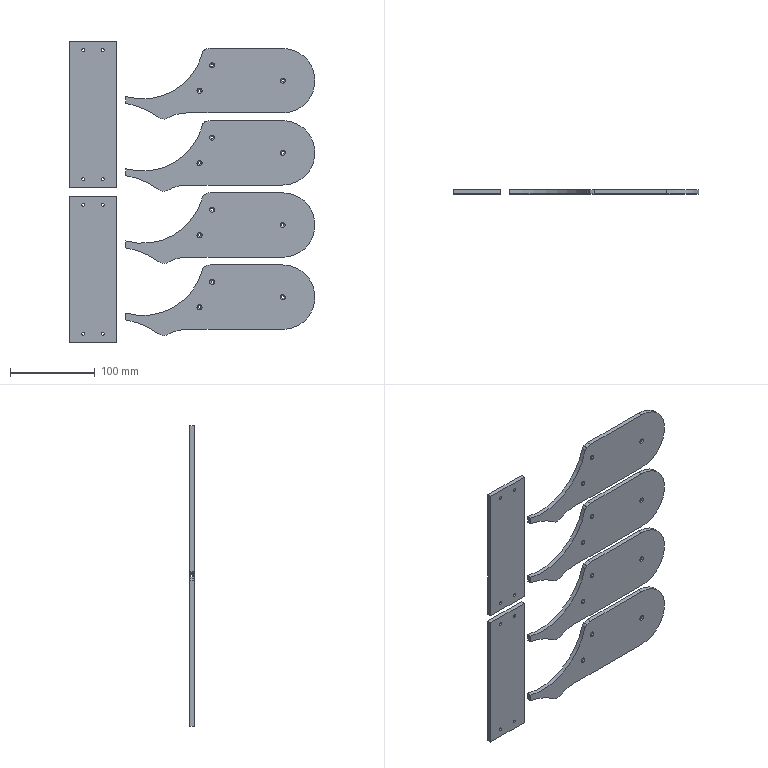CAM job | Mastercam | mm | 4 operations | part box 289.5 x 5 x 354
1. Contour (Ramp) | 3 - 3 平铣刀
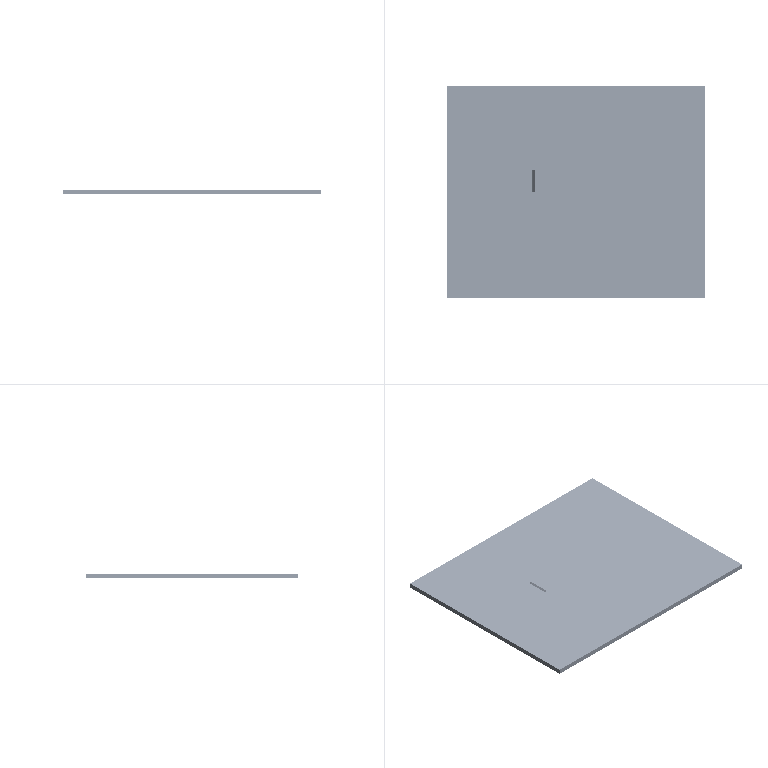2. Contour (2D) | 3 - 3 平铣刀
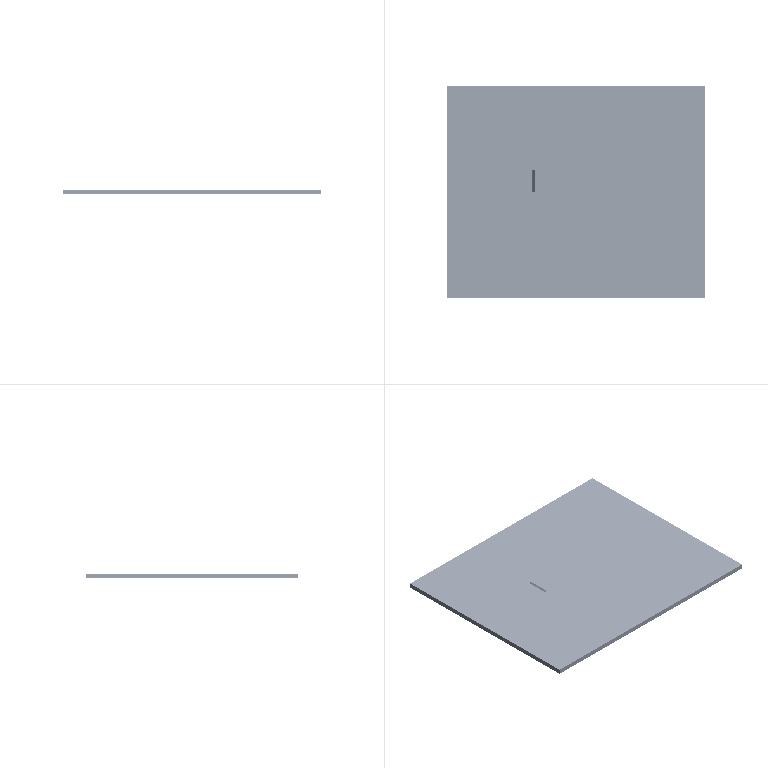3. Drill/Counterbore | 7 - 4 倒角刀
4. Contour (2D chamfer) | 7 - 4 倒角刀